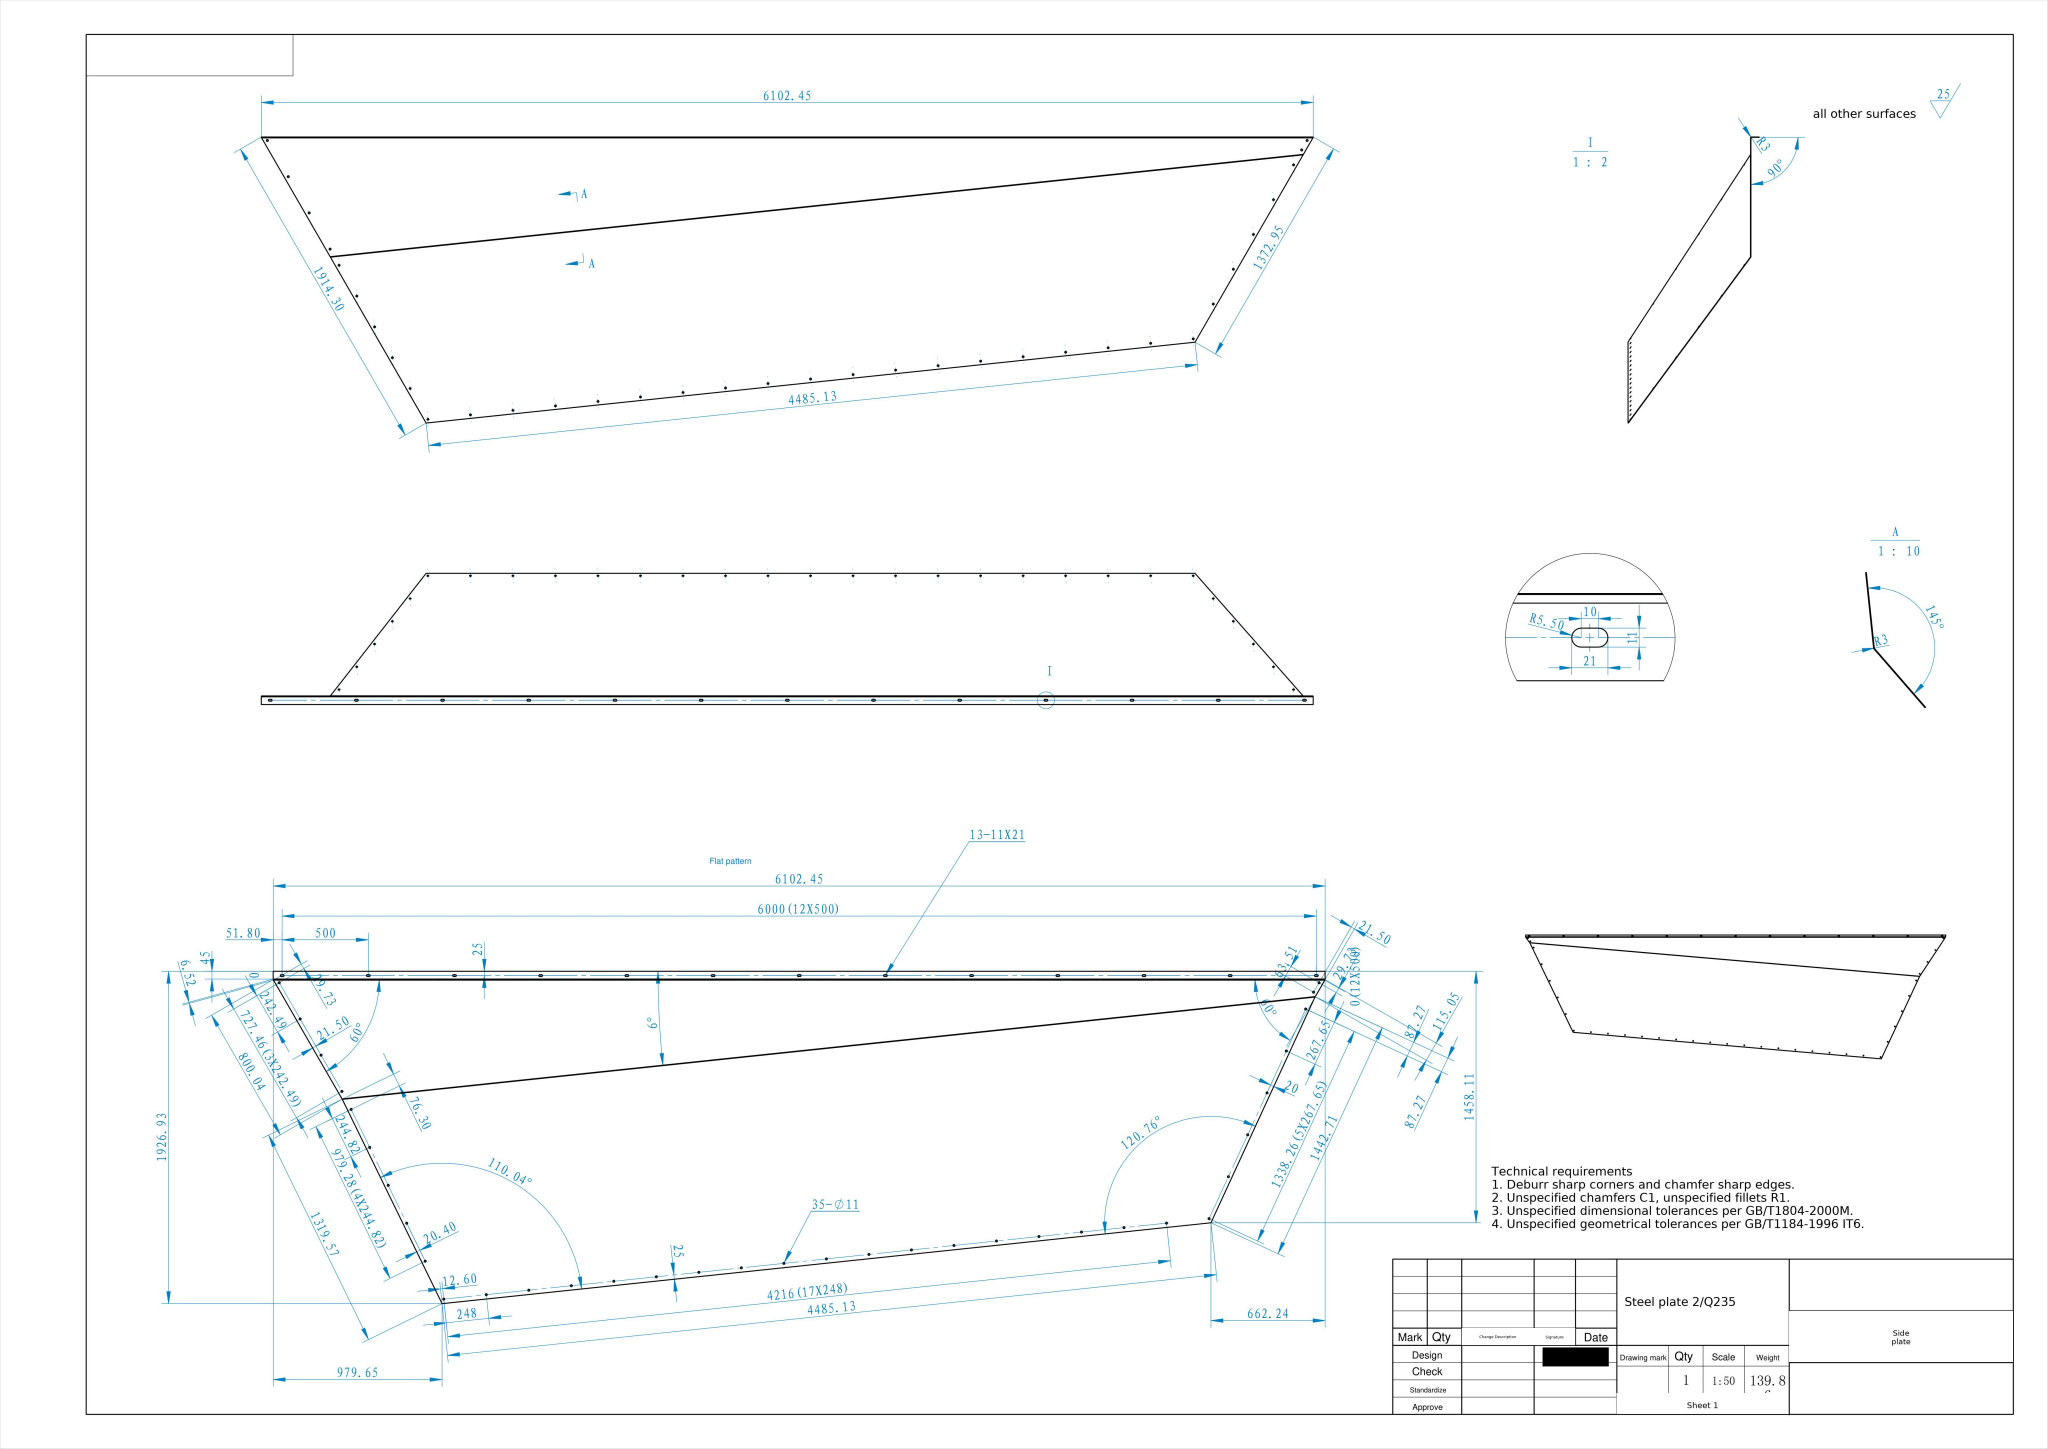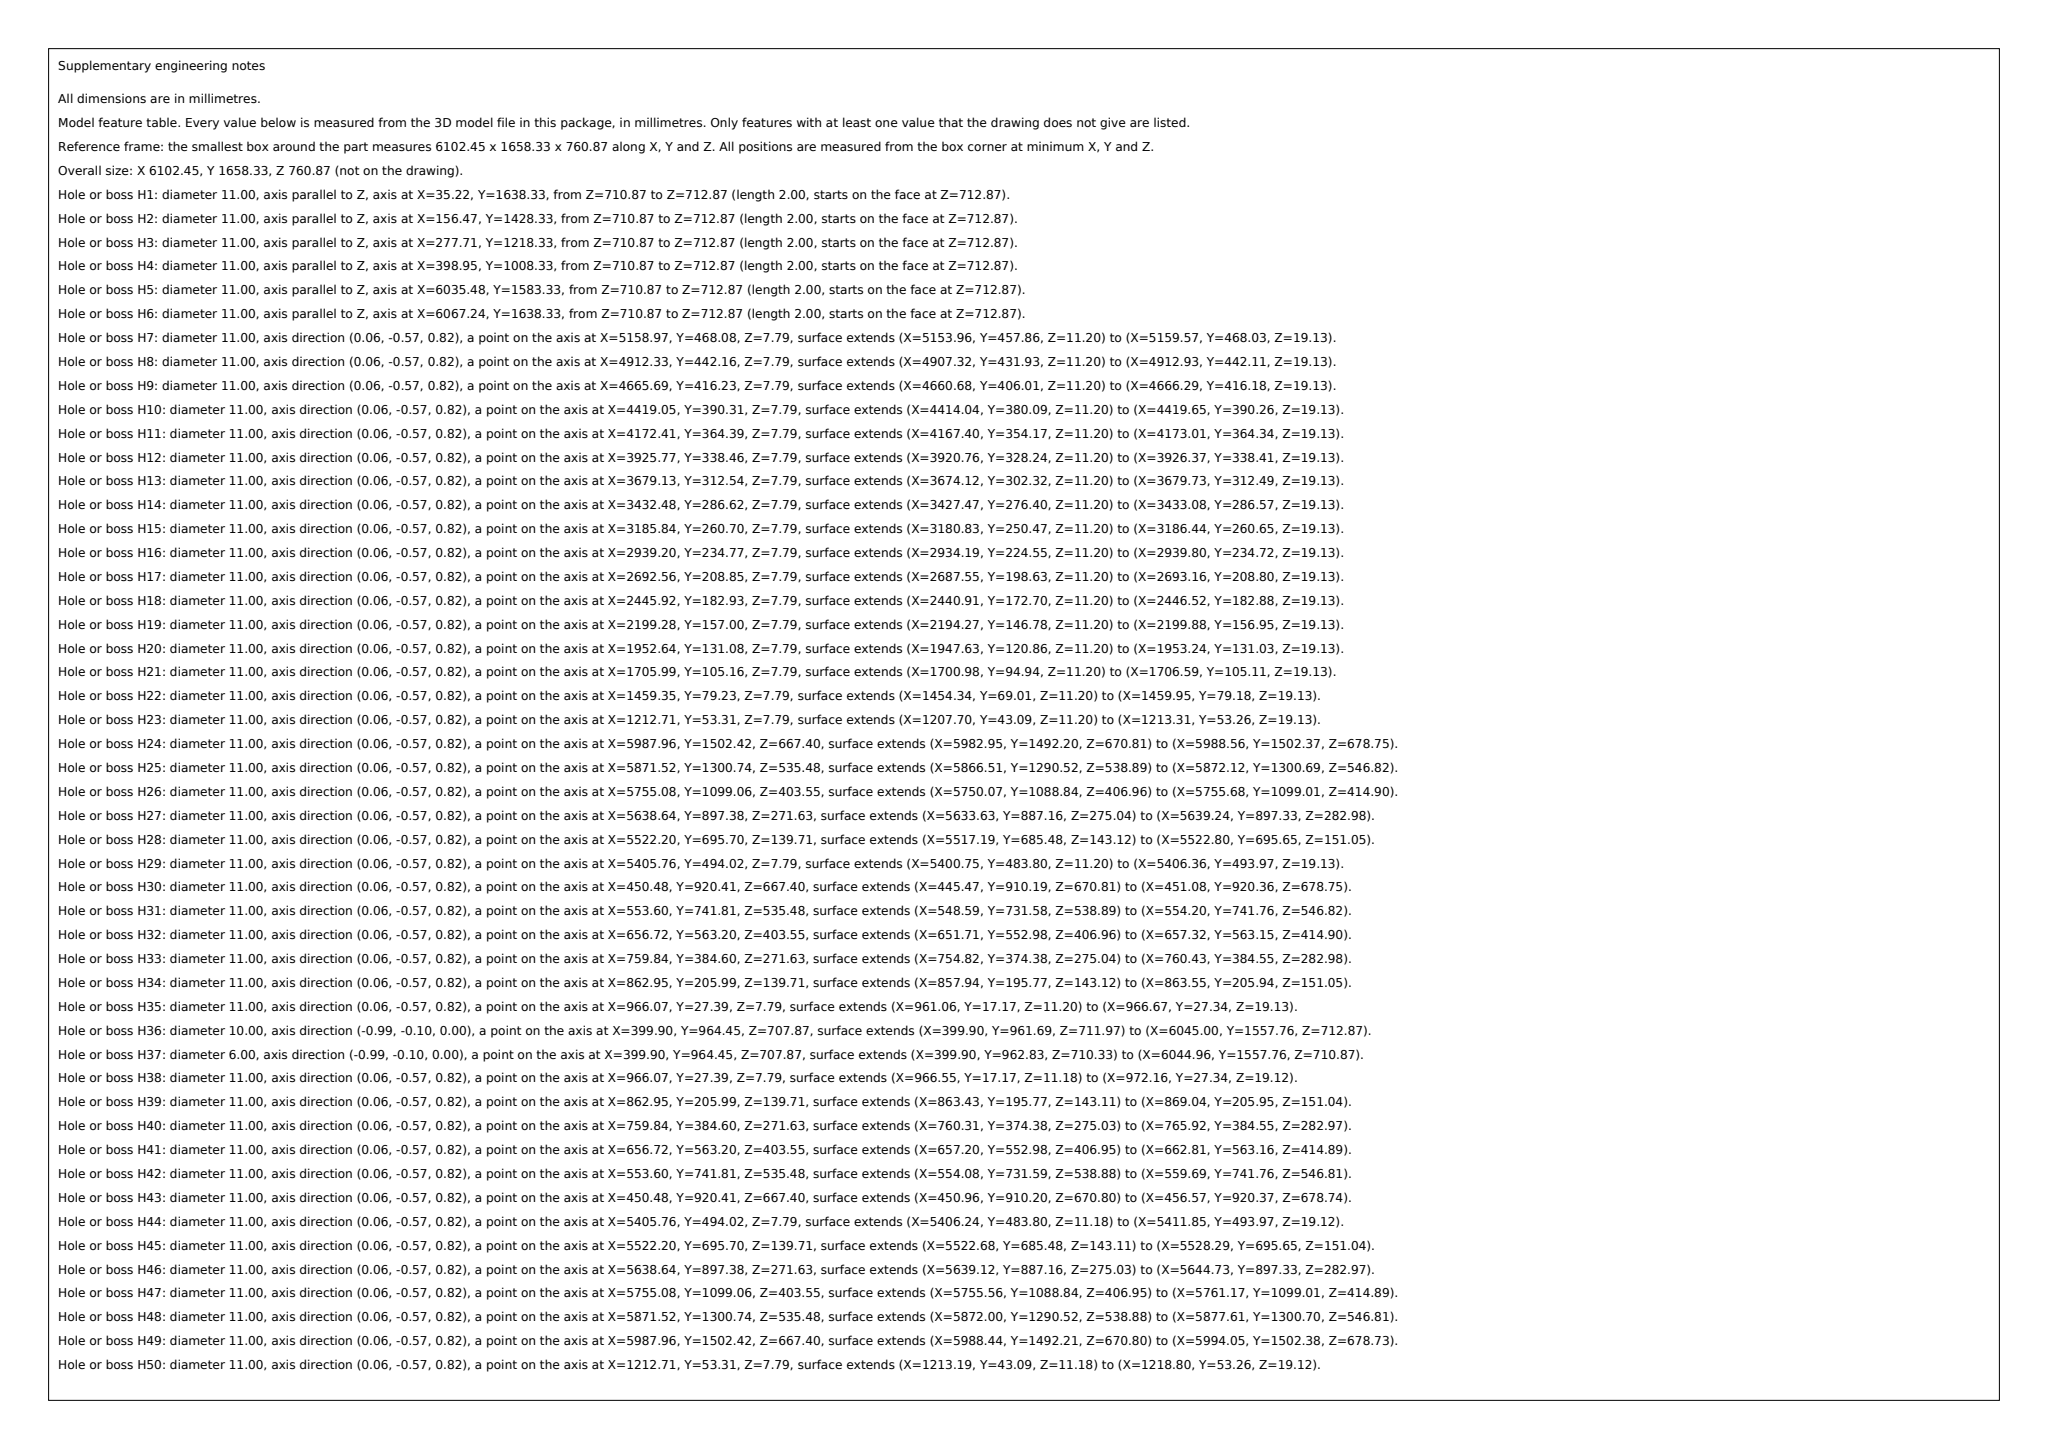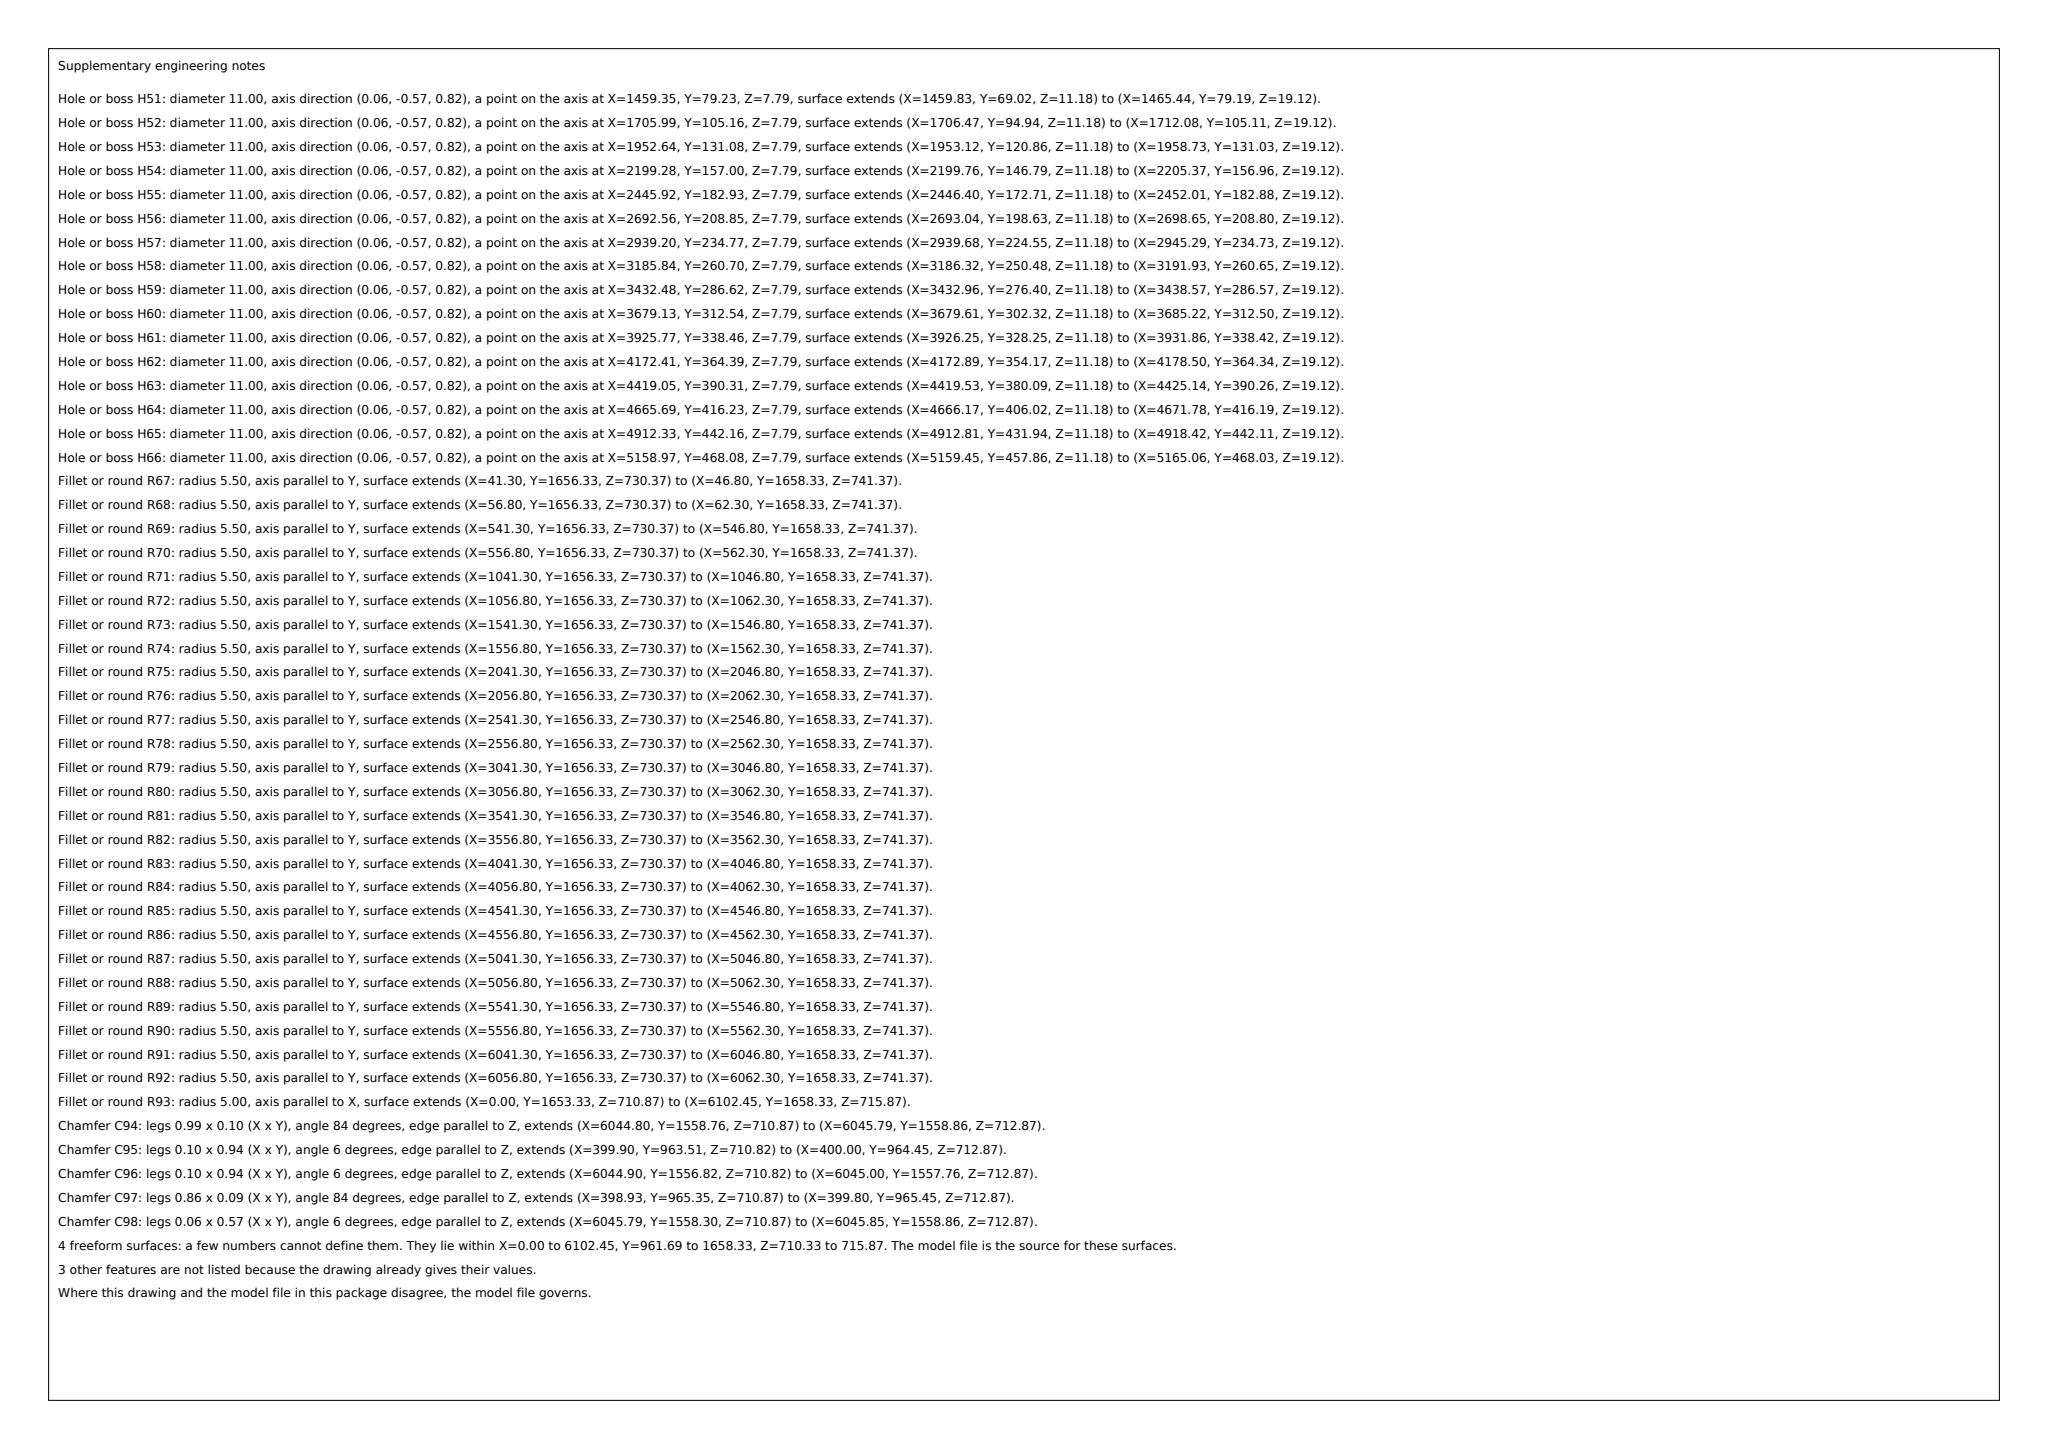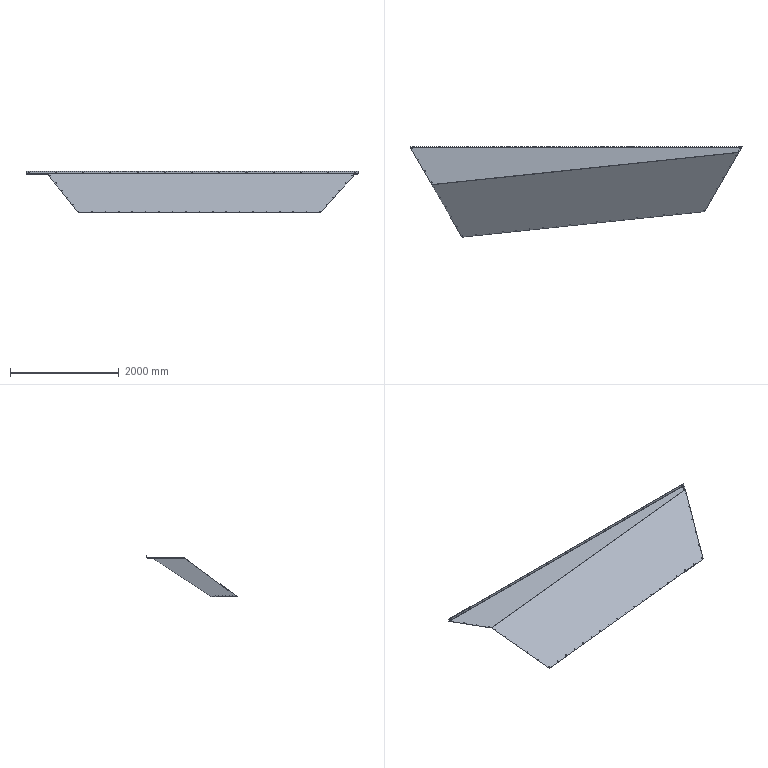Part | SolidWorks | mm | material Steel plate 2/Q235 | 1 solid | 151 faces | box 6102.45 x 1658.33 x 760.87 mm | volume 17930940 mm3 | cylinder 100 | plane 47 | spline 4 | commonest cylinder face diameters 11 x96 10 x2 6 x2